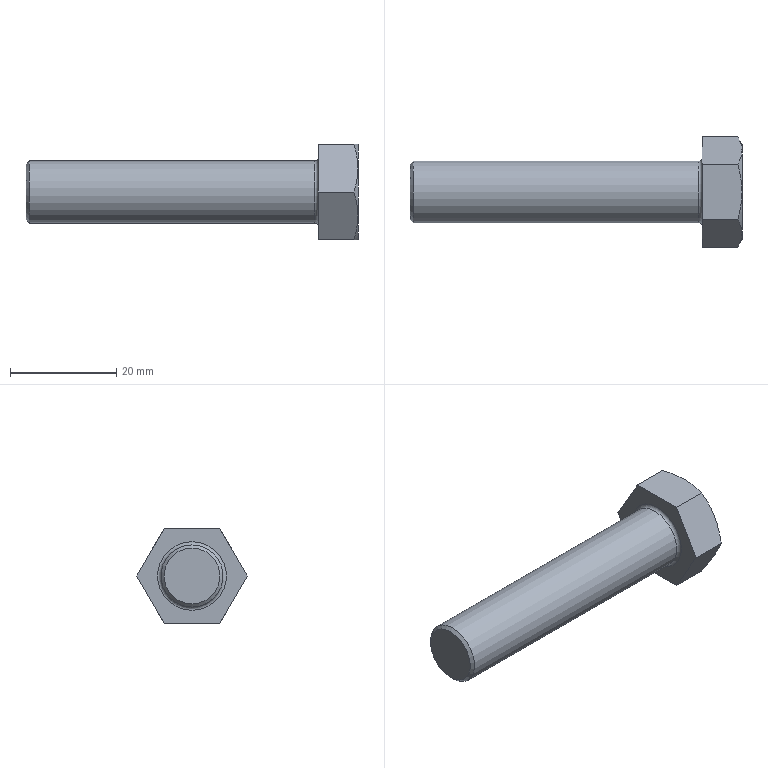Component | NX | GB-T5780-2000_M12X55 | 1 solid | 18 faces | volume 8009 mm3 | plane 9 | cone 7 | cylinder 1 | torus 1 | commonest cylinder face diameters 11.701 x1